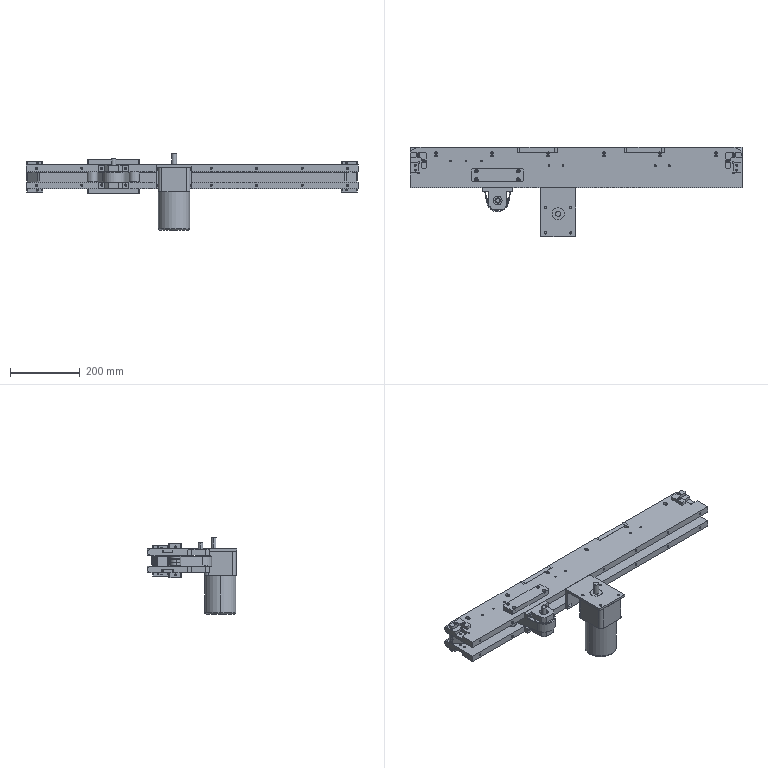Assembly | SolidWorks | mm | 73 component files | 73 solids | 1723 faces | box 950 x 255 x 218 mm | volume 6229019 mm3 | cylinder 660 | plane 581 | torus 418 | cone 64 | commonest cylinder face diameters 5 x116 10 x92 4.2 x64 8 x64 12 x48 16 x45 6 x40 8.5 x40
Bill of materials:
'--MA18S2004110mmSolderingIron | 2 |  | Long slender solid cylindrical rod with a shallow flat (D-shaped cut) on one side, where the flat appears to be interrupted along an intermediate length segment.
'--MA18S20041115GU-50KB90W | 1 |  | Motor-like body: a square housing with rounded corners on top of a cylindrical can. A short round boss and a protruding cylindrical shaft sit on the square face, which has four small holes near its corners.
'--MA18S2004111xlMotorMountOutline2 | 1 |  | L-shaped angle bracket made from constant-thickness plate. The horizontal leg has a large central circular hole and four small holes on a square pattern; the vertical leg has four elongated slots.
'--MA18S200416000Bearing | 4 |  | Annular ring with a rectangular cross-section and rounded edges. Concentric grooves on both faces mark separate inner and outer rings with a recessed annular face between them, which looks like a sealed or shielded ball bearing.
'--MA18S200416201Bearing | 2 |  | Annular ring like the previous bearing-shaped part: a short cylinder with a central bore and concentric face grooves at the inner and outer edges of the face, which look like the boundaries of a shielded ball bearing.
'--MA18S20041688Bearing | 20 |  | Annular ring with a larger bore relative to its outside diameter than the other bearing-shaped parts. It has several concentric grooves on the face and rounded edges, consistent with a thin-section shielded bearing.
'--MA18S200418mmSolderingIron | 4 |  | Long slender solid cylindrical rod with a shallow flat (D-shaped cut) on one side, apparently interrupted over a middle length segment; it looks very similar to unnamed part.
'--MA18S20041AxisStopBlock1 | 4 |  | Thick flat L-shaped (corner) plate with chamfered outer corners, a chamfered inside corner, and one round through-hole in each leg.
'--MA18S20041JR-SHuangGWAdjustingFixingBlock1 | 2 |  | Rectangular bar or plate with chamfered corners, four through-holes in pairs near each end, and one small hole in one end face.
'--MA18S20041JR-SHuangGWAdjustingRoller | 2 |  | Thin-walled plain cylindrical tube or sleeve, open at both ends with a constant wall thickness.
'--MA18S20041JR-SHuangGWBearingHousing1 | 2 |  | T-shaped block: a rectangular crossbar with a stem that has chamfered end corners. A large stepped (counterbored) round hole goes through the stem, and a small cross-hole runs through each end of the crossbar.
'--MA18S20041JR-SHuangGWBelt1 | 1 |  | Very thin-walled closed band that follows a long bar-shaped outline, with angled ends and a short tapered tab with a rounded end on one side. It appears to be only a shell or outline wall with an empty interior.
'--MA18S20041JR-SHuangGWDriveWheel | 1 |  | Short solid cylindrical disc with a smaller-diameter coaxial pin through its center. The pin sticks out from both faces, much further on one side than the other, and there is a thin stepped collar where the pin meets each face.
'--MA18S20041JR-SHuangGWGasket1 | 20 |  | Thin, flat annular ring (washer-like) with a large central through-hole and plain cylindrical inner and outer edges.
'--MA18S20041JR-SHuangGWGasket2 | 4 |  | Plain annular ring or short tube segment, noticeably thicker axially than unnamed part, with a central through-bore and flat parallel end faces.
'--MA18S20041JR-SHuangGWSupportPlate2 | 1 |  | Long, slender straight bar of rectangular cross-section with angled or chamfered ends and a row of six small, evenly spaced holes along one narrow face.
'--MA18S20041SidePlate1 | 1 |  | Long, flat rectangular plate with many small holes scattered across its face, one long elongated slot near one end, a row of holes along one side edge, chamfered corners, and a stepped notch cut into one end.
'--MA18S20041SidePlate2 | 1 |  | Long, flat rectangular plate that looks very similar to unnamed part, with a long slot near one end, side-edge holes and chamfered corners. It differs in having stepped notches at both ends and a different hole pattern on the face, including larger holes that may be counterbored along the plate.
Mates:
1. parallel | --MA18S20041SidePlate1-1 face at (-177.956, 118.699, 19) dir (0, 1, 0) | --MA18S200418mmSolderingIron-1 face at (-160.377, 99.699, 53) dir (0, 1, 0)
2. concentric | --MA18S200418mmSolderingIron-1 face at (-165.956, 96.699, 68) dir (0, 0, -1) r 4 | --MA18S20041JR-SHuangGWGasket1-1 face at (-165.956, 96.699, 19.5) dir (0, 0, -1) r 4.25
3. coincident | --MA18S20041SidePlate1-1 face at (-177.956, 118.699, 19) dir (0, 0, 1) | --MA18S20041JR-SHuangGWGasket1-1 face at (-165.956, 96.699, 19) dir (0, 0, -1)
4. concentric | --MA18S200418mmSolderingIron-1 face at (-165.956, 96.699, 68) dir (0, 0, -1) r 4 | --MA18S20041688Bearing-1 face at (-165.956, 96.699, 24.5) dir (0, 0, 1) r 4
5. coincident | --MA18S20041JR-SHuangGWGasket1-1 face at (-165.956, 96.699, 19.5) dir (0, 0, 1) | --MA18S20041688Bearing-1 face at (-164.878, 103.362, 19.5) dir (0, 0, -1)
6. coincident | --MA18S200418mmSolderingIron-1 face at (-165.956, 96.699, 68) dir (0, 0, 1) | --MA18S200418mmSolderingIron-17 face at (-137.956, 66.699, 68) dir (0, 0, 1)
7. concentric | --MA18S200418mmSolderingIron-17 face at (-137.956, 66.699, 68) dir (0, 0, -1) r 4 | --MA18S20041JR-SHuangGWGasket1-258 edge at (-137.956, 66.699, 19) dir (0, 0, 1) r 4.25
8. coincident | --MA18S20041SidePlate1-1 face at (-177.956, 118.699, 19) dir (0, 0, 1) | --MA18S20041JR-SHuangGWGasket1-258 edge at (-137.956, 66.699, 19) dir (0, 0, 1) r 6
9. concentric | --MA18S200418mmSolderingIron-17 face at (-137.956, 66.699, 68) dir (0, 0, -1) r 4 | --MA18S20041688Bearing-258 face at (-137.956, 66.699, 24.5) dir (0, 0, 1) r 4
10. coincident | --MA18S20041688Bearing-258 face at (-131.206, 66.699, 19.5) dir (0, 0, -1) | --MA18S20041JR-SHuangGWGasket1-258 face at (-137.956, 66.699, 19.5) dir (0, 0, 1)
11. coincident | --MA18S200418mmSolderingIron-19 face at (732.044, 66.699, 68) dir (0, 0, 1) | --MA18S200418mmSolderingIron-20 face at (760.044, 96.699, 68) dir (0, 0, 1)
12. coincident | --MA18S200418mmSolderingIron-17 face at (-137.956, 66.699, 68) dir (0, 0, 1) | --MA18S200418mmSolderingIron-19 face at (732.044, 66.699, 68) dir (0, 0, 1)
13. coincident | --MA18S20041JR-SHuangGWGasket1-295 face at (760.044, 96.699, 19) dir (0, 0, -1) | --MA18S20041JR-SHuangGWGasket1-300 face at (732.044, 66.699, 19) dir (0, 0, -1)
14. coincident | --MA18S20041SidePlate1-1 face at (-177.956, 118.699, 19) dir (0, 0, 1) | --MA18S20041JR-SHuangGWGasket1-295 face at (760.044, 96.699, 19) dir (0, 0, -1)
15. concentric | --MA18S200418mmSolderingIron-20 face at (760.044, 96.699, 68) dir (0, 0, -1) r 4 | --MA18S20041JR-SHuangGWGasket1-295 face at (760.044, 96.699, 19.5) dir (0, 0, -1) r 4.25
16. concentric | --MA18S200418mmSolderingIron-19 face at (732.044, 66.699, 68) dir (0, 0, -1) r 4 | --MA18S20041JR-SHuangGWGasket1-300 face at (732.044, 66.699, 19.5) dir (0, 0, -1) r 4.25
17. concentric | --MA18S200418mmSolderingIron-19 face at (732.044, 66.699, 68) dir (0, 0, -1) r 4 | --MA18S20041688Bearing-300 face at (732.044, 66.699, 24.5) dir (0, 0, 1) r 4
18. coincident | --MA18S200418mmSolderingIron-20 face at (760.044, 96.699, 68) dir (0, 0, -1) r 4 | --MA18S20041688Bearing-295 edge at (760.044, 96.699, 24) dir (0, 0, 1) r 4
19. coincident | --MA18S20041688Bearing-295 face at (754.232, 93.267, 24.5) dir (0, 0, 1) | --MA18S20041688Bearing-300 face at (738.794, 66.699, 24.5) dir (0, 0, 1)
20. coincident | --MA18S20041688Bearing-258 face at (-131.206, 66.699, 24.5) dir (0, 0, 1) | --MA18S20041688Bearing-300 face at (738.794, 66.699, 24.5) dir (0, 0, 1)
21. coincident | --MA18S200416201Bearing-1 face at (86.048, -27.843, 8) dir (0, 0, -1) | --MA18S20041JR-SHuangGWBearingHousing1-1 edge at (72.885, -33.301, 8) dir (0, 0, 1) r 16
22. concentric | --MA18S200416201Bearing-1 face at (72.885, -33.301, 18) dir (0, 0, 1) r 6 | --MA18S20041JR-SHuangGWBearingHousing1-1 face at (72.885, -33.301, 1) dir (0, 0, 1) r 12.5
23. coincident | --MA18S20041SidePlate1-1 face at (-177.956, 3.699, 19) dir (0, -1, 0) | --MA18S20041JR-SHuangGWBearingHousing1-1 face at (115.885, 3.699, 1) dir (0, 1, 0)
24. coincident | --MA18S200416201Bearing-1 face at (86.048, -27.843, 18) dir (0, 0, 1) | --MA18S20041JR-SHuangGWDriveWheel-1 face at (72.885, -33.301, 18) dir (0, 0, -1)
25. concentric | --MA18S200416201Bearing-1 face at (72.885, -33.301, 18) dir (0, 0, 1) r 6 | --MA18S20041JR-SHuangGWDriveWheel-1 face at (72.885, -33.301, 7) dir (0, 0, 1) r 6
26. coincident | --MA18S20041JR-SHuangGWAdjustingRoller-1 face at (12.044, 38.699, 39) dir (0, 0, 1) | --MA18S200416000Bearing-2 face at (23.294, 38.699, 39) dir (0, 0, -1)
27. concentric | --MA18S20041JR-SHuangGWAdjustingRoller-1 face at (12.044, 38.699, 39) dir (0, 0, 1) r 13 | --MA18S200416000Bearing-2 face at (12.044, 38.699, 47) dir (0, 0, 1) r 13
28. concentric | --MA18S200416000Bearing-1 face at (12.044, 38.699, 29) dir (0, 0, 1) r 13 | --MA18S20041JR-SHuangGWAdjustingRoller-1 face at (12.044, 38.699, 29) dir (0, 0, -1) r 13
29. coincident | --MA18S200416000Bearing-1 face at (23.294, 38.699, 29) dir (0, 0, 1) | --MA18S20041JR-SHuangGWAdjustingRoller-1 face at (12.044, 38.699, 29) dir (0, 0, -1)
30. concentric | --MA18S200416000Bearing-2 face at (12.044, 38.699, 47) dir (0, 0, 1) r 5 | --MA18S2004110mmSolderingIron-1 face at (12.044, 38.699, 78) dir (0, 0, -1) r 5
31. distance | --MA18S2004110mmSolderingIron-1 face at (12.044, 38.699, -10) dir (0, 0, -1) | --MA18S20041JR-SHuangGWAdjustingRoller-1 face at (12.044, 38.699, 20) dir (0, 0, -1)
32. distance | --MA18S20041JR-SHuangGWAdjustingRoller-1 face at (12.044, 38.699, 20) dir (0, 0, -1) | --MA18S20041SidePlate1-1 face at (-177.956, 118.699, 19) dir (0, 0, 1)
33. coincident | --MA18S200416000Bearing-3 face at (143.294, 38.699, 29) dir (0, 0, 1) | --MA18S20041JR-SHuangGWAdjustingRoller-2 edge at (132.044, 38.699, 29) dir (0, 0, -1) r 12
34. concentric | --MA18S200416000Bearing-3 face at (132.044, 38.699, 21) dir (0, 0, -1) r 13 | --MA18S20041JR-SHuangGWAdjustingRoller-2 face at (132.044, 38.699, 48) dir (0, 0, -1) r 15
35. coincident | --MA18S200416000Bearing-4 face at (143.294, 38.699, 39) dir (0, 0, -1) | --MA18S20041JR-SHuangGWAdjustingRoller-2 face at (132.044, 38.699, 39) dir (0, 0, 1)
36. concentric | --MA18S200416000Bearing-4 face at (132.044, 38.699, 39) dir (0, 0, -1) r 13 | --MA18S20041JR-SHuangGWAdjustingRoller-2 face at (132.044, 38.699, 39) dir (0, 0, 1) r 13
37. concentric | --MA18S200416000Bearing-4 face at (132.044, 38.699, 39) dir (0, 0, -1) r 5 | --MA18S2004110mmSolderingIron-2 face at (132.044, 38.699, -10) dir (0, 0, 1) r 5
38. coincident | --MA18S2004110mmSolderingIron-1 face at (12.044, 38.699, 78) dir (0, 0, 1) | --MA18S2004110mmSolderingIron-2 face at (132.044, 38.699, 78) dir (0, 0, 1)
39. coincident | --MA18S20041JR-SHuangGWAdjustingRoller-1 face at (12.044, 38.699, 48) dir (0, 0, 1) | --MA18S20041JR-SHuangGWAdjustingRoller-2 face at (132.044, 38.699, 48) dir (0, 0, 1)
40. coincident | --MA18S20041SidePlate1-1 face at (-177.956, 118.699, 19) dir (0, 1, 0) | --MA18S20041SidePlate2-1 face at (-177.956, 118.699, 68) dir (0, 1, 0)
41. coincident | --MA18S20041SidePlate2-1 face at (-177.956, 3.699, 68) dir (0, -1, 0) | --MA18S20041JR-SHuangGWBearingHousing1-2 face at (29.885, 3.699, 67.5) dir (0, 1, 0)
42. concentric | --MA18S20041SidePlate2-1 face at (38.885, 3.699, 58) dir (0, -1, 0) r 3 | --MA18S20041JR-SHuangGWBearingHousing1-2 face at (38.885, -8.301, 58) dir (0, -1, 0) r 3.25
43. coincident | --MA18S20041JR-SHuangGWBearingHousing1-2 face at (72.885, -33.301, 60.5) dir (0, 0, -1) | --MA18S200416201Bearing-2 face at (87.135, -33.301, 60.5) dir (0, 0, 1)
44. concentric | --MA18S20041JR-SHuangGWBearingHousing1-2 face at (72.885, -33.301, 60.5) dir (0, 0, -1) r 16 | --MA18S200416201Bearing-2 face at (72.885, -33.301, 60.5) dir (0, 0, 1) r 16
45. distance | --MA18S20041SidePlate2-1 face at (-177.956, 118.699, 49) dir (0, 0, -1) | --MA18S20041SidePlate1-1 face at (-177.956, 118.699, 19) dir (0, 0, 1)
46. coincident | --MA18S20041SidePlate1-1 face at (-177.956, 118.699, 19) dir (0, 0, 1) | --MA18S20041JR-SHuangGWSupportPlate2-1 face at (-142.956, 93.699, 19) dir (0, 0, -1)
47. distance | --MA18S20041JR-SHuangGWSupportPlate2-1 face at (-142.956, 103.699, 19) dir (0, 1, 0) | --MA18S20041SidePlate1-1 face at (-177.956, 118.699, 19) dir (0, 1, 0)
48. distance | --MA18S20041JR-SHuangGWSupportPlate2-1 face at (-142.956, 93.699, 49) dir (-1, 0, 0) | --MA18S20041SidePlate1-1 face at (-177.956, 3.699, 19) dir (-1, 0, 0)
49. coincident | --MA18S20041SidePlate1-1 face at (-177.956, 118.699, 19) dir (0, 0, 1) | --MA18S20041JR-SHuangGWBelt1-1 face at (760.044, 96.699, 19) dir (0, 0, -1)
50. coincident | --MA18S20041SidePlate2-1 face at (-177.956, 118.699, 68) dir (0, 0, 1) | --MA18S20041JR-SHuangGWAdjustingFixingBlock1-1 face at (-2.956, 57.199, 68) dir (0, 0, -1)
51. coincident | --MA18S20041SidePlate1-1 face at (-177.956, 118.699, 0) dir (0, 0, -1) | --MA18S20041JR-SHuangGWAdjustingFixingBlock1-2 face at (147.044, 57.199, 0) dir (0, 0, 1)
52. coincident | --MA18S20041JR-SHuangGWAdjustingFixingBlock1-1 face at (-2.956, 57.199, 83) dir (0, 1, 0) | --MA18S20041JR-SHuangGWAdjustingFixingBlock1-2 face at (147.044, 57.199, -15) dir (0, 1, 0)
53. coincident | --MA18S20041JR-SHuangGWAdjustingFixingBlock1-1 face at (-2.956, 20.199, 83) dir (-1, 0, 0) | --MA18S20041JR-SHuangGWAdjustingFixingBlock1-2 face at (-2.956, 20.199, -15) dir (-1, 0, 0)
54. concentric | --MA18S2004110mmSolderingIron-1 face at (12.044, 38.699, 78) dir (0, 0, -1) r 5 | --MA18S20041JR-SHuangGWGasket2-1 face at (12.044, 38.699, 19) dir (0, 0, 1) r 5
55. coincident | --MA18S200416000Bearing-1 face at (18.294, 38.699, 21) dir (0, 0, -1) | --MA18S20041JR-SHuangGWGasket2-1 face at (12.044, 38.699, 21) dir (0, 0, 1)
56. concentric | --MA18S2004110mmSolderingIron-2 face at (132.044, 38.699, -10) dir (0, 0, 1) r 5 | --MA18S20041JR-SHuangGWGasket2-4 face at (132.044, 38.699, 47) dir (0, 0, 1) r 5
57. concentric | --MA18S20041SidePlate1-1 face at (12.044, 38.699, -131.461) dir (0, 0, 1) r 5.5 | --MA18S2004110mmSolderingIron-1 face at (12.044, 38.699, 78) dir (0, 0, -1) r 5
58. concentric | --MA18S2004110mmSolderingIron-2 face at (132.044, 38.699, -10) dir (0, 0, 1) r 5 | --MA18S20041SidePlate2-1 face at (132.044, 38.699, 49) dir (0, 0, 1) r 5.5
59. concentric | --MA18S200418mmSolderingIron-20 face at (760.044, 96.699, 68) dir (0, 0, -1) r 4 | --MA18S20041SidePlate2-1 face at (760.044, 96.699, 68) dir (0, 0, -1) r 4
60. coincident | --MA18S200418mmSolderingIron-17 face at (-137.956, 66.699, 68) dir (0, 0, 1) | --MA18S20041SidePlate2-1 face at (-177.956, 118.699, 68) dir (0, 0, 1)
61. concentric | --MA18S200418mmSolderingIron-19 face at (732.044, 66.699, 68) dir (0, 0, -1) r 4 | --MA18S20041SidePlate2-1 face at (732.044, 66.699, 68) dir (0, 0, -1) r 4
62. concentric | --MA18S200418mmSolderingIron-1 face at (-165.956, 96.699, 68) dir (0, 0, -1) r 4 | --MA18S20041SidePlate2-1 face at (-165.956, 96.699, 68) dir (0, 0, -1) r 4
63. concentric | --MA18S200418mmSolderingIron-17 face at (-137.956, 66.699, 68) dir (0, 0, -1) r 4 | --MA18S20041SidePlate2-1 face at (-137.956, 66.699, 68) dir (0, 0, -1) r 4
64. coincident | --MA18S20041SidePlate1-1 face at (12.044, 33.199, -131.461) dir (0, 1, 0) | --MA18S20041JR-SHuangGWAdjustingFixingBlock1-2 face at (7.044, 33.199, -10) dir (0, 1, 0)
65. distance | --MA18S20041JR-SHuangGWAdjustingFixingBlock1-2 face at (-2.956, 20.199, -15) dir (-1, 0, 0) | --MA18S20041SidePlate1-1 face at (-177.956, 3.699, 19) dir (-1, 0, 0)
66. coincident | --MA18S20041SidePlate2-1 face at (-177.956, 3.699, 68) dir (0, -1, 0) | --MA18S2004111xlMotorMountOutline2-1 face at (295.885, 3.699, 68) dir (0, 1, 0)
67. coincident | --MA18S20041SidePlate2-1 face at (-177.956, 118.699, 68) dir (0, 0, 1) | --MA18S2004111xlMotorMountOutline2-1 face at (295.885, 3.699, 68) dir (0, 0, 1)
68. distance | --MA18S2004111xlMotorMountOutline2-1 face at (195.885, 3.699, 0) dir (-1, 0, 0) | --MA18S20041JR-SHuangGWBearingHousing1-2 face at (115.885, 3.699, 49.5) dir (1, 0, 0)
69. concentric | --MA18S20041115GU-50KB90W-1 face at (245.885, -71.301, 99.5) dir (0, 0, -1) r 7.5 | --MA18S2004111xlMotorMountOutline2-1 face at (245.885, -71.301, 0) dir (0, 0, 1) r 17.5
70. coincident | --MA18S20041115GU-50KB90W-1 face at (200.885, -134.801, 61) dir (0, 0, 1) | --MA18S2004111xlMotorMountOutline2-1 face at (295.885, -136.301, 61) dir (0, 0, -1)
71. coincident | --MA18S20041SidePlate2-1 face at (-177.956, 118.699, 68) dir (0, 0, 1) | --MA18S20041AxisStopBlock1-1 face at (-145.456, 59.199, 68) dir (0, 0, -1)
72. distance | --MA18S20041AxisStopBlock1-1 face at (-175.456, 104.199, 77.5) dir (0, 1, 0) | --MA18S20041SidePlate2-1 face at (-177.956, 118.699, 68) dir (0, 1, 0)
73. distance | --MA18S20041AxisStopBlock1-1 face at (-175.456, 89.199, 77.5) dir (-1, 0, 0) | --MA18S20041SidePlate2-1 face at (-177.956, 3.699, 68) dir (-1, 0, 0)
74. coincident | --MA18S20041AxisStopBlock1-1 face at (-145.456, 59.199, 77.5) dir (0, 0, 1) | --MA18S20041AxisStopBlock1-2 face at (769.544, 89.199, 77.5) dir (0, 0, 1)
75. coincident | --MA18S20041AxisStopBlock1-1 face at (-175.456, 104.199, 77.5) dir (0, 1, 0) | --MA18S20041AxisStopBlock1-2 face at (724.544, 104.199, 77.5) dir (0, 1, 0)
76. distance | --MA18S20041AxisStopBlock1-2 face at (769.544, 104.199, 77.5) dir (1, 0, 0) | --MA18S20041SidePlate2-1 face at (772.044, 3.699, 68) dir (1, 0, 0)
77. coincident | --MA18S20041SidePlate1-1 face at (-177.956, 118.699, 0) dir (0, 0, -1) | --MA18S20041AxisStopBlock1-3 face at (-175.456, 89.199, 0) dir (0, 0, 1)
78. coincident | --MA18S20041AxisStopBlock1-1 face at (-175.456, 104.199, 77.5) dir (0, 1, 0) | --MA18S20041AxisStopBlock1-3 face at (-130.456, 104.199, -9.5) dir (0, 1, 0)
79. coincident | --MA18S20041AxisStopBlock1-1 face at (-175.456, 89.199, 77.5) dir (-1, 0, 0) | --MA18S20041AxisStopBlock1-3 face at (-175.456, 104.199, -9.5) dir (-1, 0, 0)
80. coincident | --MA18S20041SidePlate1-1 face at (-177.956, 118.699, 0) dir (0, 0, -1) | --MA18S20041AxisStopBlock1-4 face at (739.544, 59.199, 0) dir (0, 0, 1)
81. coincident | --MA18S20041AxisStopBlock1-2 face at (724.544, 104.199, 77.5) dir (0, 1, 0) | --MA18S20041AxisStopBlock1-4 face at (769.544, 104.199, -9.5) dir (0, 1, 0)
82. coincident | --MA18S20041AxisStopBlock1-2 face at (724.544, 59.199, 77.5) dir (-1, 0, 0) | --MA18S20041AxisStopBlock1-4 face at (724.544, 104.199, -9.5) dir (-1, 0, 0)
83. concentric | --MA18S20041SidePlate1-1 face at (38.885, 3.699, 10.5) dir (0, -1, 0) r 3 | --MA18S20041JR-SHuangGWBearingHousing1-1 face at (38.885, -8.301, 10.5) dir (0, -1, 0) r 3.25
84. concentric | --MA18S200418mmSolderingIron-20 face at (760.044, 96.699, 68) dir (0, 0, -1) r 4 | --MA18S20041JR-SHuangGWBelt1-1 face at (760.044, 96.699, 47) dir (0, 0, -1) r 8
85. parallel | --MA18S20041SidePlate1-1 face at (-177.956, 118.699, 19) dir (0, 1, 0) | --MA18S20041JR-SHuangGWBelt1-1 face at (-165.956, 106.699, 47) dir (0, 1, 0)